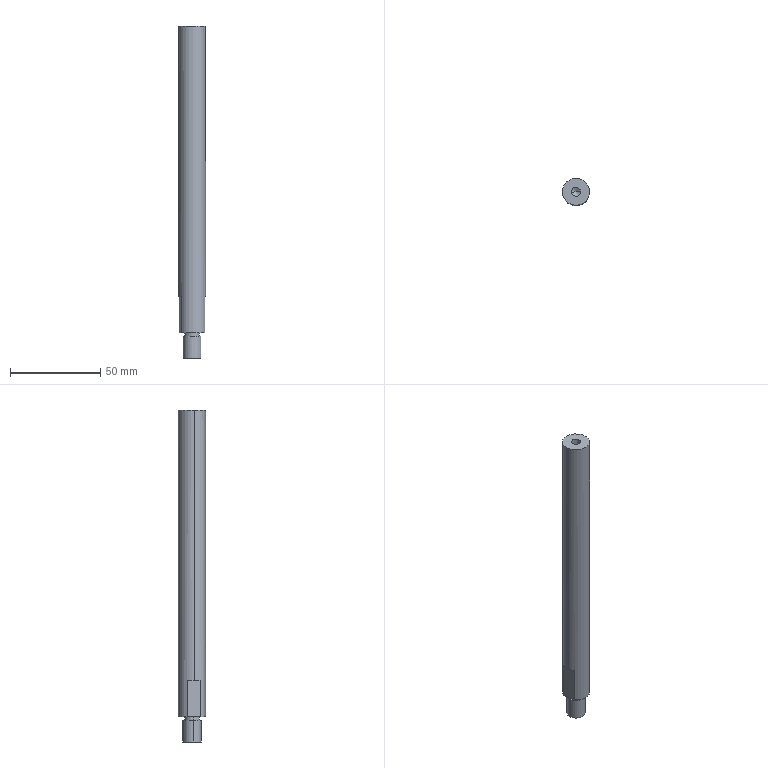Component | SolidWorks | -CoverTopPost-1 | 1 solid | 18 faces | box 15 x 15 x 184 mm | volume 30538 mm3 | cylinder 8 | plane 8 | cone 2 | commonest cylinder face diameters 10 x2 8 x2 5 x2 15 x2
build123d program:
from build123d import *

# Parameters (mm, degrees)
SKETCH1_R             = 7.5
BOSS_EXTRUDE1_DEPTH   = 85
M6_TAPPED_HOLE1_D     = 5
M6_TAPPED_HOLE1_DEPTH = 17
M6_TAPPED_HOLE1_TIP   = 1.502
SKETCH4_R             = 4
BOSS_EXTRUDE2_DEPTH   = 2
SKETCH5_R             = 5
BOSS_EXTRUDE3_DEPTH   = 12
SKETCH6_W             = 19.221
SKETCH6_H             = 36.695
SKETCH6_W_2           = 15.818
SKETCH6_H_2           = 41.018
CUT_EXTRUDE1_DEPTH    = 20


with BuildPart() as part:
    # Sketch1 → Boss-Extrude1 (new, symmetric)
    with BuildSketch(Plane.XY):
        Circle(SKETCH1_R)
    extrude(amount=BOSS_EXTRUDE1_DEPTH, both=True)

    # M6 Tapped Hole1
    with Locations(Plane.XY.offset(85)):
        with Locations((0, 0)):
            Hole(M6_TAPPED_HOLE1_D / 2, depth=M6_TAPPED_HOLE1_DEPTH)
            with Locations((0, 0, -(M6_TAPPED_HOLE1_DEPTH + M6_TAPPED_HOLE1_TIP / 2))):  # 118° drill point
                Cone(0, M6_TAPPED_HOLE1_D / 2, M6_TAPPED_HOLE1_TIP, mode=Mode.SUBTRACT)

    # Sketch4 → Boss-Extrude2 (add)
    with BuildSketch(Plane(origin=(0, 0, -85), x_dir=(-1, 0, 0), z_dir=(0, 0, -1))):
        with Locations(Location((0, 0, 0), (0, 0, 180))):
            Circle(SKETCH4_R)
    extrude(amount=BOSS_EXTRUDE2_DEPTH)

    # Sketch5 → Boss-Extrude3 (add)
    with BuildSketch(Plane(origin=(0, 0, -87), x_dir=(-1, 0, 0), z_dir=(0, 0, -1))):
        Circle(SKETCH5_R)
    extrude(amount=BOSS_EXTRUDE3_DEPTH)

    # Sketch6 → Cut-Extrude1 (cut)
    with BuildSketch(Plane(origin=(0, 0, -85), x_dir=(-1, 0, 0), z_dir=(0, 0, -1))):
        with Locations((-16.111, -0.5037)):
            Rectangle(SKETCH6_W, SKETCH6_H)
        with Locations((14.409, -0.5497)):
            Rectangle(SKETCH6_W_2, SKETCH6_H_2)
    extrude(amount=-CUT_EXTRUDE1_DEPTH, mode=Mode.SUBTRACT)


solid = part.part

# Placed as in the assembly
solid = solid.moved(Location((-15, 1079.5, 90), (0, 0, 9.293)))
STEP:
#1=COLOUR_RGB('',0.7922,0.8196,0.9333);
#2=FILL_AREA_STYLE_COLOUR('',#1);
#3=FILL_AREA_STYLE('',(#2));
#4=SURFACE_STYLE_FILL_AREA(#3);
#5=SURFACE_SIDE_STYLE('',(#4));
#6=SURFACE_STYLE_USAGE(.BOTH.,#5);
#7=PRESENTATION_STYLE_ASSIGNMENT((#6));
#8=CARTESIAN_POINT('',(-0.7848,42.468,-0.3543));
#9=VERTEX_POINT('',#8);
#10=CARTESIAN_POINT('',(-0.3963,42.532,-0.3543));
#11=VERTEX_POINT('',#10);
#12=CARTESIAN_POINT('',(-0.5906,42.5,-0.3543));
#13=DIRECTION('',(0.,0.,-1.));
#14=DIRECTION('',(-0.9869,-0.1615,0.));
#15=AXIS2_PLACEMENT_3D('',#12,#13,#14);
#16=CIRCLE('',#15,0.1969);
#17=EDGE_CURVE('',#9,#11,#16,.T.);
#18=ORIENTED_EDGE('',*,*,#17,.F.);
#19=CARTESIAN_POINT('',(-0.7848,42.468,0.1181));
#20=VERTEX_POINT('',#19);
#21=CARTESIAN_POINT('',(-0.7848,42.468,-0.3543));
#22=DIRECTION('',(0.,0.,1.));
#23=VECTOR('',#22,39.37);
#24=LINE('',#21,#23);
#25=EDGE_CURVE('',#9,#20,#24,.T.);
#26=ORIENTED_EDGE('',*,*,#25,.T.);
#27=CARTESIAN_POINT('',(-0.3963,42.532,0.1181));
#28=VERTEX_POINT('',#27);
#29=CARTESIAN_POINT('',(-0.5906,42.5,0.1181));
#30=DIRECTION('',(0.,0.,-1.));
#31=DIRECTION('',(-0.9869,-0.1615,0.));
#32=AXIS2_PLACEMENT_3D('',#29,#30,#31);
#33=CIRCLE('',#32,0.1969);
#34=EDGE_CURVE('',#20,#28,#33,.T.);
#35=ORIENTED_EDGE('',*,*,#34,.T.);
#36=CARTESIAN_POINT('',(-0.3963,42.532,-0.3543));
#37=DIRECTION('',(0.,0.,1.));
#38=VECTOR('',#37,39.37);
#39=LINE('',#36,#38);
#40=EDGE_CURVE('',#11,#28,#39,.T.);
#41=ORIENTED_EDGE('',*,*,#40,.F.);
#42=EDGE_LOOP('',(#18,#26,#35,#41));
#43=FACE_OUTER_BOUND('',#42,.T.);
#44=CARTESIAN_POINT('',(-0.5906,42.5,-0.3543));
#45=DIRECTION('',(0.,0.,1.));
#46=DIRECTION('',(0.9869,0.1615,0.));
#47=AXIS2_PLACEMENT_3D('',#44,#45,#46);
#48=CYLINDRICAL_SURFACE('',#47,0.1969);
#49=ADVANCED_FACE('',(#43),#48,.T.);
#50=CARTESIAN_POINT('',(-0.746,42.475,0.1181));
#51=VERTEX_POINT('',#50);
#52=CARTESIAN_POINT('',(-0.4351,42.525,0.1181));
#53=VERTEX_POINT('',#52);
#54=CARTESIAN_POINT('',(-0.5906,42.5,0.1181));
#55=DIRECTION('',(0.,0.,-1.));
#56=DIRECTION('',(-0.9869,-0.1615,0.));
#57=AXIS2_PLACEMENT_3D('',#54,#55,#56);
#58=CIRCLE('',#57,0.1575);
#59=EDGE_CURVE('',#51,#53,#58,.T.);
#60=ORIENTED_EDGE('',*,*,#59,.F.);
#61=CARTESIAN_POINT('',(-0.746,42.475,0.1969));
#62=VERTEX_POINT('',#61);
#63=CARTESIAN_POINT('',(-0.746,42.475,0.1181));
#64=DIRECTION('',(0.,0.,1.));
#65=VECTOR('',#64,39.37);
#66=LINE('',#63,#65);
#67=EDGE_CURVE('',#51,#62,#66,.T.);
#68=ORIENTED_EDGE('',*,*,#67,.T.);
#69=CARTESIAN_POINT('',(-0.4351,42.525,0.1969));
#70=VERTEX_POINT('',#69);
#71=CARTESIAN_POINT('',(-0.5906,42.5,0.1969));
#72=DIRECTION('',(0.,0.,-1.));
#73=DIRECTION('',(0.9869,0.1615,0.));
#74=AXIS2_PLACEMENT_3D('',#71,#72,#73);
#75=CIRCLE('',#74,0.1575);
#76=EDGE_CURVE('',#62,#70,#75,.T.);
#77=ORIENTED_EDGE('',*,*,#76,.T.);
#78=CARTESIAN_POINT('',(-0.4351,42.525,0.1181));
#79=DIRECTION('',(0.,0.,1.));
#80=VECTOR('',#79,39.37);
#81=LINE('',#78,#80);
#82=EDGE_CURVE('',#53,#70,#81,.T.);
#83=ORIENTED_EDGE('',*,*,#82,.F.);
#84=EDGE_LOOP('',(#60,#68,#77,#83));
#85=FACE_OUTER_BOUND('',#84,.T.);
#86=CARTESIAN_POINT('',(-0.5906,42.5,0.1181));
#87=DIRECTION('',(0.,0.,1.));
#88=DIRECTION('',(0.9869,0.1615,0.));
#89=AXIS2_PLACEMENT_3D('',#86,#87,#88);
#90=CYLINDRICAL_SURFACE('',#89,0.1575);
#91=ADVANCED_FACE('',(#85),#90,.T.);
#92=CARTESIAN_POINT('',(-0.6877,42.484,6.22));
#93=VERTEX_POINT('',#92);
#94=CARTESIAN_POINT('',(-0.4934,42.516,6.22));
#95=VERTEX_POINT('',#94);
#96=CARTESIAN_POINT('',(-0.5906,42.5,6.22));
#97=DIRECTION('',(0.,0.,1.));
#98=DIRECTION('',(0.9869,0.1615,0.));
#99=AXIS2_PLACEMENT_3D('',#96,#97,#98);
#100=CIRCLE('',#99,0.09843);
#101=EDGE_CURVE('',#93,#95,#100,.T.);
#102=ORIENTED_EDGE('',*,*,#101,.F.);
#103=CARTESIAN_POINT('',(-0.6877,42.484,6.89));
#104=VERTEX_POINT('',#103);
#105=CARTESIAN_POINT('',(-0.6877,42.484,6.89));
#106=DIRECTION('',(0.,0.,1.));
#107=VECTOR('',#106,39.37);
#108=LINE('',#105,#107);
#109=EDGE_CURVE('',#93,#104,#108,.T.);
#110=ORIENTED_EDGE('',*,*,#109,.T.);
#111=CARTESIAN_POINT('',(-0.4934,42.516,6.89));
#112=VERTEX_POINT('',#111);
#113=CARTESIAN_POINT('',(-0.5906,42.5,6.89));
#114=DIRECTION('',(0.,0.,1.));
#115=DIRECTION('',(0.9869,0.1615,0.));
#116=AXIS2_PLACEMENT_3D('',#113,#114,#115);
#117=CIRCLE('',#116,0.09843);
#118=EDGE_CURVE('',#104,#112,#117,.T.);
#119=ORIENTED_EDGE('',*,*,#118,.T.);
#120=CARTESIAN_POINT('',(-0.4934,42.516,6.89));
#121=DIRECTION('',(0.,0.,1.));
#122=VECTOR('',#121,39.37);
#123=LINE('',#120,#122);
#124=EDGE_CURVE('',#95,#112,#123,.T.);
#125=ORIENTED_EDGE('',*,*,#124,.F.);
#126=EDGE_LOOP('',(#102,#110,#119,#125));
#127=FACE_OUTER_BOUND('',#126,.T.);
#128=CARTESIAN_POINT('',(-0.5906,42.5,6.89));
#129=DIRECTION('',(0.,0.,1.));
#130=DIRECTION('',(0.9869,0.1615,0.));
#131=AXIS2_PLACEMENT_3D('',#128,#129,#130);
#132=CYLINDRICAL_SURFACE('',#131,0.09843);
#133=ADVANCED_FACE('',(#127),#132,.F.);
#134=CARTESIAN_POINT('',(-0.5906,42.5,6.161));
#135=VERTEX_POINT('',#134);
#136=CARTESIAN_POINT('',(-0.4934,42.516,6.22));
#137=DIRECTION('',(0.8459,0.1384,0.515));
#138=VECTOR('',#137,39.37);
#139=LINE('',#136,#138);
#140=EDGE_CURVE('',#135,#95,#139,.T.);
#141=ORIENTED_EDGE('',*,*,#140,.F.);
#142=CARTESIAN_POINT('',(-0.6877,42.484,6.22));
#143=DIRECTION('',(-0.8459,-0.1384,0.515));
#144=VECTOR('',#143,39.37);
#145=LINE('',#142,#144);
#146=EDGE_CURVE('',#135,#93,#145,.T.);
#147=ORIENTED_EDGE('',*,*,#146,.T.);
#148=ORIENTED_EDGE('',*,*,#101,.T.);
#149=EDGE_LOOP('',(#141,#147,#148));
#150=FACE_OUTER_BOUND('',#149,.T.);
#151=CARTESIAN_POINT('',(-0.5906,42.5,6.22));
#152=DIRECTION('',(0.,0.,1.));
#153=DIRECTION('',(0.9869,0.1615,0.));
#154=AXIS2_PLACEMENT_3D('',#151,#152,#153);
#155=CONICAL_SURFACE('',#154,0.09843,1.03);
#156=ADVANCED_FACE('',(#150),#155,.F.);
#157=CARTESIAN_POINT('',(-0.2992,42.548,6.89));
#158=VERTEX_POINT('',#157);
#159=CARTESIAN_POINT('',(-0.882,42.452,6.89));
#160=VERTEX_POINT('',#159);
#161=CARTESIAN_POINT('',(-0.5906,42.5,6.89));
#162=DIRECTION('',(0.,0.,1.));
#163=DIRECTION('',(0.9869,0.1615,0.));
#164=AXIS2_PLACEMENT_3D('',#161,#162,#163);
#165=CIRCLE('',#164,0.2953);
#166=EDGE_CURVE('',#158,#160,#165,.T.);
#167=ORIENTED_EDGE('',*,*,#166,.F.);
#168=CARTESIAN_POINT('',(-0.2992,42.548,0.9843));
#169=VERTEX_POINT('',#168);
#170=CARTESIAN_POINT('',(-0.2992,42.548,6.89));
#171=DIRECTION('',(0.,0.,-1.));
#172=VECTOR('',#171,39.37);
#173=LINE('',#170,#172);
#174=EDGE_CURVE('',#158,#169,#173,.T.);
#175=ORIENTED_EDGE('',*,*,#174,.T.);
#176=CARTESIAN_POINT('',(-0.3618,42.687,0.9843));
#177=VERTEX_POINT('',#176);
#178=CARTESIAN_POINT('',(-0.5906,42.5,0.9843));
#179=DIRECTION('',(0.,0.,-1.));
#180=DIRECTION('',(-0.9869,-0.1615,0.));
#181=AXIS2_PLACEMENT_3D('',#178,#179,#180);
#182=CIRCLE('',#181,0.2953);
#183=EDGE_CURVE('',#177,#169,#182,.T.);
#184=ORIENTED_EDGE('',*,*,#183,.F.);
#185=CARTESIAN_POINT('',(-0.3618,42.687,0.1969));
#186=VERTEX_POINT('',#185);
#187=CARTESIAN_POINT('',(-0.3618,42.687,6.89));
#188=DIRECTION('',(0.,0.,-1.));
#189=VECTOR('',#188,39.37);
#190=LINE('',#187,#189);
#191=EDGE_CURVE('',#177,#186,#190,.T.);
#192=ORIENTED_EDGE('',*,*,#191,.T.);
#193=CARTESIAN_POINT('',(-0.8669,42.604,0.1969));
#194=VERTEX_POINT('',#193);
#195=CARTESIAN_POINT('',(-0.5906,42.5,0.1969));
#196=DIRECTION('',(0.,0.,1.));
#197=DIRECTION('',(0.9869,0.1615,0.));
#198=AXIS2_PLACEMENT_3D('',#195,#196,#197);
#199=CIRCLE('',#198,0.2953);
#200=EDGE_CURVE('',#186,#194,#199,.T.);
#201=ORIENTED_EDGE('',*,*,#200,.T.);
#202=CARTESIAN_POINT('',(-0.8669,42.604,0.9843));
#203=VERTEX_POINT('',#202);
#204=CARTESIAN_POINT('',(-0.8669,42.604,6.89));
#205=DIRECTION('',(0.,0.,1.));
#206=VECTOR('',#205,39.37);
#207=LINE('',#204,#206);
#208=EDGE_CURVE('',#194,#203,#207,.T.);
#209=ORIENTED_EDGE('',*,*,#208,.T.);
#210=CARTESIAN_POINT('',(-0.882,42.452,0.9843));
#211=VERTEX_POINT('',#210);
#212=CARTESIAN_POINT('',(-0.5906,42.5,0.9843));
#213=DIRECTION('',(0.,0.,1.));
#214=DIRECTION('',(0.9869,0.1615,0.));
#215=AXIS2_PLACEMENT_3D('',#212,#213,#214);
#216=CIRCLE('',#215,0.2953);
#217=EDGE_CURVE('',#203,#211,#216,.T.);
#218=ORIENTED_EDGE('',*,*,#217,.T.);
#219=CARTESIAN_POINT('',(-0.882,42.452,6.89));
#220=DIRECTION('',(0.,0.,-1.));
#221=VECTOR('',#220,39.37);
#222=LINE('',#219,#221);
#223=EDGE_CURVE('',#160,#211,#222,.T.);
#224=ORIENTED_EDGE('',*,*,#223,.F.);
#225=EDGE_LOOP('',(#167,#175,#184,#192,#201,#209,#218,#224));
#226=FACE_OUTER_BOUND('',#225,.T.);
#227=CARTESIAN_POINT('',(-0.5906,42.5,6.89));
#228=DIRECTION('',(0.,0.,-1.));
#229=DIRECTION('',(-0.9869,-0.1615,0.));
#230=AXIS2_PLACEMENT_3D('',#227,#228,#229);
#231=CYLINDRICAL_SURFACE('',#230,0.2953);
#232=ADVANCED_FACE('',(#226),#231,.T.);
#233=CARTESIAN_POINT('',(-0.8193,42.313,0.1969));
#234=VERTEX_POINT('',#233);
#235=CARTESIAN_POINT('',(-0.3142,42.396,0.1969));
#236=VERTEX_POINT('',#235);
#237=CARTESIAN_POINT('',(-0.5906,42.5,0.1969));
#238=DIRECTION('',(0.,0.,1.));
#239=DIRECTION('',(0.9869,0.1615,0.));
#240=AXIS2_PLACEMENT_3D('',#237,#238,#239);
#241=CIRCLE('',#240,0.2953);
#242=EDGE_CURVE('',#234,#236,#241,.T.);
#243=ORIENTED_EDGE('',*,*,#242,.F.);
#244=CARTESIAN_POINT('',(-0.97,43.234,0.1969));
#245=DIRECTION('',(0.1615,-0.9869,0.));
#246=VECTOR('',#245,39.37);
#247=LINE('',#244,#246);
#248=EDGE_CURVE('',#194,#234,#247,.T.);
#249=ORIENTED_EDGE('',*,*,#248,.F.);
#250=ORIENTED_EDGE('',*,*,#200,.F.);
#251=CARTESIAN_POINT('',(-0.4514,43.235,0.1969));
#252=DIRECTION('',(-0.1615,0.9869,0.));
#253=VECTOR('',#252,39.37);
#254=LINE('',#251,#253);
#255=EDGE_CURVE('',#236,#186,#254,.T.);
#256=ORIENTED_EDGE('',*,*,#255,.F.);
#257=EDGE_LOOP('',(#243,#249,#250,#256));
#258=FACE_OUTER_BOUND('',#257,.T.);
#259=CARTESIAN_POINT('',(-0.5906,42.5,0.1969));
#260=DIRECTION('',(0.,0.,-1.));
#261=DIRECTION('',(0.9869,0.1615,0.));
#262=AXIS2_PLACEMENT_3D('',#259,#260,#261);
#263=CIRCLE('',#262,0.1575);
#264=EDGE_CURVE('',#70,#62,#263,.T.);
#265=ORIENTED_EDGE('',*,*,#264,.F.);
#266=ORIENTED_EDGE('',*,*,#76,.F.);
#267=EDGE_LOOP('',(#265,#266));
#268=FACE_BOUND('',#267,.T.);
#269=CARTESIAN_POINT('',(-0.5906,42.5,0.1969));
#270=DIRECTION('',(0.,0.,1.));
#271=DIRECTION('',(0.9869,0.1615,0.));
#272=AXIS2_PLACEMENT_3D('',#269,#270,#271);
#273=PLANE('',#272);
#274=ADVANCED_FACE('',(#258,#268),#273,.F.);
#275=ORIENTED_EDGE('',*,*,#174,.F.);
#276=CARTESIAN_POINT('',(-0.5906,42.5,6.89));
#277=DIRECTION('',(0.,0.,1.));
#278=DIRECTION('',(0.9869,0.1615,0.));
#279=AXIS2_PLACEMENT_3D('',#276,#277,#278);
#280=CIRCLE('',#279,0.2953);
#281=EDGE_CURVE('',#160,#158,#280,.T.);
#282=ORIENTED_EDGE('',*,*,#281,.F.);
#283=ORIENTED_EDGE('',*,*,#223,.T.);
#284=CARTESIAN_POINT('',(-0.8193,42.313,0.9843));
#285=VERTEX_POINT('',#284);
#286=CARTESIAN_POINT('',(-0.5906,42.5,0.9843));
#287=DIRECTION('',(0.,0.,1.));
#288=DIRECTION('',(0.9869,0.1615,0.));
#289=AXIS2_PLACEMENT_3D('',#286,#287,#288);
#290=CIRCLE('',#289,0.2953);
#291=EDGE_CURVE('',#211,#285,#290,.T.);
#292=ORIENTED_EDGE('',*,*,#291,.T.);
#293=CARTESIAN_POINT('',(-0.8193,42.313,6.89));
#294=DIRECTION('',(0.,0.,-1.));
#295=VECTOR('',#294,39.37);
#296=LINE('',#293,#295);
#297=EDGE_CURVE('',#285,#234,#296,.T.);
#298=ORIENTED_EDGE('',*,*,#297,.T.);
#299=ORIENTED_EDGE('',*,*,#242,.T.);
#300=CARTESIAN_POINT('',(-0.3142,42.396,0.9843));
#301=VERTEX_POINT('',#300);
#302=CARTESIAN_POINT('',(-0.3142,42.396,6.89));
#303=DIRECTION('',(0.,0.,1.));
#304=VECTOR('',#303,39.37);
#305=LINE('',#302,#304);
#306=EDGE_CURVE('',#236,#301,#305,.T.);
#307=ORIENTED_EDGE('',*,*,#306,.T.);
#308=CARTESIAN_POINT('',(-0.5906,42.5,0.9843));
#309=DIRECTION('',(0.,0.,-1.));
#310=DIRECTION('',(-0.9869,-0.1615,0.));
#311=AXIS2_PLACEMENT_3D('',#308,#309,#310);
#312=CIRCLE('',#311,0.2953);
#313=EDGE_CURVE('',#169,#301,#312,.T.);
#314=ORIENTED_EDGE('',*,*,#313,.F.);
#315=EDGE_LOOP('',(#275,#282,#283,#292,#298,#299,#307,#314));
#316=FACE_OUTER_BOUND('',#315,.T.);
#317=CARTESIAN_POINT('',(-0.5906,42.5,6.89));
#318=DIRECTION('',(0.,0.,-1.));
#319=DIRECTION('',(-0.9869,-0.1615,0.));
#320=AXIS2_PLACEMENT_3D('',#317,#318,#319);
#321=CYLINDRICAL_SURFACE('',#320,0.2953);
#322=ADVANCED_FACE('',(#316),#321,.T.);
#323=CARTESIAN_POINT('',(-0.5906,42.5,6.89));
#324=DIRECTION('',(0.,0.,1.));
#325=DIRECTION('',(0.9869,0.1615,0.));
#326=AXIS2_PLACEMENT_3D('',#323,#324,#325);
#327=CIRCLE('',#326,0.09843);
#328=EDGE_CURVE('',#112,#104,#327,.T.);
#329=ORIENTED_EDGE('',*,*,#328,.F.);
#330=ORIENTED_EDGE('',*,*,#118,.F.);
#331=EDGE_LOOP('',(#329,#330));
#332=FACE_BOUND('',#331,.T.);
#333=ORIENTED_EDGE('',*,*,#281,.T.);
#334=ORIENTED_EDGE('',*,*,#166,.T.);
#335=EDGE_LOOP('',(#333,#334));
#336=FACE_OUTER_BOUND('',#335,.T.);
#337=CARTESIAN_POINT('',(-0.5906,42.5,6.89));
#338=DIRECTION('',(0.,0.,1.));
#339=DIRECTION('',(0.9869,0.1615,0.));
#340=AXIS2_PLACEMENT_3D('',#337,#338,#339);
#341=PLANE('',#340);
#342=ADVANCED_FACE('',(#332,#336),#341,.T.);
#343=ORIENTED_EDGE('',*,*,#146,.F.);
#344=ORIENTED_EDGE('',*,*,#140,.T.);
#345=CARTESIAN_POINT('',(-0.5906,42.5,6.22));
#346=DIRECTION('',(0.,0.,1.));
#347=DIRECTION('',(0.9869,0.1615,0.));
#348=AXIS2_PLACEMENT_3D('',#345,#346,#347);
#349=CIRCLE('',#348,0.09843);
#350=EDGE_CURVE('',#95,#93,#349,.T.);
#351=ORIENTED_EDGE('',*,*,#350,.T.);
#352=EDGE_LOOP('',(#343,#344,#351));
#353=FACE_OUTER_BOUND('',#352,.T.);
#354=CARTESIAN_POINT('',(-0.5906,42.5,6.22));
#355=DIRECTION('',(0.,0.,1.));
#356=DIRECTION('',(0.9869,0.1615,0.));
#357=AXIS2_PLACEMENT_3D('',#354,#355,#356);
#358=CONICAL_SURFACE('',#357,0.09843,1.03);
#359=ADVANCED_FACE('',(#353),#358,.F.);
#360=ORIENTED_EDGE('',*,*,#109,.F.);
#361=ORIENTED_EDGE('',*,*,#350,.F.);
#362=ORIENTED_EDGE('',*,*,#124,.T.);
#363=ORIENTED_EDGE('',*,*,#328,.T.);
#364=EDGE_LOOP('',(#360,#361,#362,#363));
#365=FACE_OUTER_BOUND('',#364,.T.);
#366=CARTESIAN_POINT('',(-0.5906,42.5,6.89));
#367=DIRECTION('',(0.,0.,1.));
#368=DIRECTION('',(0.9869,0.1615,0.));
#369=AXIS2_PLACEMENT_3D('',#366,#367,#368);
#370=CYLINDRICAL_SURFACE('',#369,0.09843);
#371=ADVANCED_FACE('',(#365),#370,.F.);
#372=ORIENTED_EDGE('',*,*,#67,.F.);
#373=CARTESIAN_POINT('',(-0.5906,42.5,0.1181));
#374=DIRECTION('',(0.,0.,-1.));
#375=DIRECTION('',(-0.9869,-0.1615,0.));
#376=AXIS2_PLACEMENT_3D('',#373,#374,#375);
#377=CIRCLE('',#376,0.1575);
#378=EDGE_CURVE('',#53,#51,#377,.T.);
#379=ORIENTED_EDGE('',*,*,#378,.F.);
#380=ORIENTED_EDGE('',*,*,#82,.T.);
#381=ORIENTED_EDGE('',*,*,#264,.T.);
#382=EDGE_LOOP('',(#372,#379,#380,#381));
#383=FACE_OUTER_BOUND('',#382,.T.);
#384=CARTESIAN_POINT('',(-0.5906,42.5,0.1181));
#385=DIRECTION('',(0.,0.,1.));
#386=DIRECTION('',(0.9869,0.1615,0.));
#387=AXIS2_PLACEMENT_3D('',#384,#385,#386);
#388=CYLINDRICAL_SURFACE('',#387,0.1575);
#389=ADVANCED_FACE('',(#383),#388,.T.);
#390=CARTESIAN_POINT('',(-0.5906,42.5,0.1181));
#391=DIRECTION('',(0.,0.,-1.));
#392=DIRECTION('',(-0.9869,-0.1615,0.));
#393=AXIS2_PLACEMENT_3D('',#390,#391,#392);
#394=CIRCLE('',#393,0.1969);
#395=EDGE_CURVE('',#28,#20,#394,.T.);
#396=ORIENTED_EDGE('',*,*,#395,.F.);
#397=ORIENTED_EDGE('',*,*,#34,.F.);
#398=EDGE_LOOP('',(#396,#397));
#399=FACE_OUTER_BOUND('',#398,.T.);
#400=ORIENTED_EDGE('',*,*,#378,.T.);
#401=ORIENTED_EDGE('',*,*,#59,.T.);
#402=EDGE_LOOP('',(#400,#401));
#403=FACE_BOUND('',#402,.T.);
#404=CARTESIAN_POINT('',(-0.5906,42.5,0.1181));
#405=DIRECTION('',(0.,0.,-1.));
#406=DIRECTION('',(-0.9869,-0.1615,0.));
#407=AXIS2_PLACEMENT_3D('',#404,#405,#406);
#408=PLANE('',#407);
#409=ADVANCED_FACE('',(#399,#403),#408,.F.);
#410=ORIENTED_EDGE('',*,*,#25,.F.);
#411=CARTESIAN_POINT('',(-0.5906,42.5,-0.3543));
#412=DIRECTION('',(0.,0.,-1.));
#413=DIRECTION('',(-0.9869,-0.1615,0.));
#414=AXIS2_PLACEMENT_3D('',#411,#412,#413);
#415=CIRCLE('',#414,0.1969);
#416=EDGE_CURVE('',#11,#9,#415,.T.);
#417=ORIENTED_EDGE('',*,*,#416,.F.);
#418=ORIENTED_EDGE('',*,*,#40,.T.);
#419=ORIENTED_EDGE('',*,*,#395,.T.);
#420=EDGE_LOOP('',(#410,#417,#418,#419));
#421=FACE_OUTER_BOUND('',#420,.T.);
#422=CARTESIAN_POINT('',(-0.5906,42.5,-0.3543));
#423=DIRECTION('',(0.,0.,1.));
#424=DIRECTION('',(0.9869,0.1615,0.));
#425=AXIS2_PLACEMENT_3D('',#422,#423,#424);
#426=CYLINDRICAL_SURFACE('',#425,0.1969);
#427=ADVANCED_FACE('',(#421),#426,.T.);
#428=ORIENTED_EDGE('',*,*,#416,.T.);
#429=ORIENTED_EDGE('',*,*,#17,.T.);
#430=EDGE_LOOP('',(#428,#429));
#431=FACE_OUTER_BOUND('',#430,.T.);
#432=CARTESIAN_POINT('',(-0.5906,42.5,-0.3543));
#433=DIRECTION('',(0.,0.,-1.));
#434=DIRECTION('',(-0.9869,-0.1615,0.));
#435=AXIS2_PLACEMENT_3D('',#432,#433,#434);
#436=PLANE('',#435);
#437=ADVANCED_FACE('',(#431),#436,.T.);
#438=CARTESIAN_POINT('',(-0.4514,43.235,0.9843));
#439=DIRECTION('',(-0.1615,0.9869,0.));
#440=VECTOR('',#439,39.37);
#441=LINE('',#438,#440);
#442=EDGE_CURVE('',#301,#177,#441,.T.);
#443=ORIENTED_EDGE('',*,*,#442,.F.);
#444=ORIENTED_EDGE('',*,*,#306,.F.);
#445=ORIENTED_EDGE('',*,*,#255,.T.);
#446=ORIENTED_EDGE('',*,*,#191,.F.);
#447=EDGE_LOOP('',(#443,#444,#445,#446));
#448=FACE_OUTER_BOUND('',#447,.T.);
#449=CARTESIAN_POINT('',(-0.4514,43.235,0.9843));
#450=DIRECTION('',(-0.9869,-0.1615,0.));
#451=DIRECTION('',(0.1615,-0.9869,0.));
#452=AXIS2_PLACEMENT_3D('',#449,#450,#451);
#453=PLANE('',#452);
#454=ADVANCED_FACE('',(#448),#453,.F.);
#455=ORIENTED_EDGE('',*,*,#183,.T.);
#456=ORIENTED_EDGE('',*,*,#313,.T.);
#457=ORIENTED_EDGE('',*,*,#442,.T.);
#458=EDGE_LOOP('',(#455,#456,#457));
#459=FACE_OUTER_BOUND('',#458,.T.);
#460=CARTESIAN_POINT('',(-0.5906,42.5,0.9843));
#461=DIRECTION('',(0.,0.,-1.));
#462=DIRECTION('',(-0.9869,-0.1615,0.));
#463=AXIS2_PLACEMENT_3D('',#460,#461,#462);
#464=PLANE('',#463);
#465=ADVANCED_FACE('',(#459),#464,.T.);
#466=CARTESIAN_POINT('',(-0.97,43.234,0.9843));
#467=DIRECTION('',(0.1615,-0.9869,0.));
#468=VECTOR('',#467,39.37);
#469=LINE('',#466,#468);
#470=EDGE_CURVE('',#203,#285,#469,.T.);
#471=ORIENTED_EDGE('',*,*,#470,.F.);
#472=ORIENTED_EDGE('',*,*,#208,.F.);
#473=ORIENTED_EDGE('',*,*,#248,.T.);
#474=ORIENTED_EDGE('',*,*,#297,.F.);
#475=EDGE_LOOP('',(#471,#472,#473,#474));
#476=FACE_OUTER_BOUND('',#475,.T.);
#477=CARTESIAN_POINT('',(-0.97,43.234,0.9843));
#478=DIRECTION('',(0.9869,0.1615,0.));
#479=DIRECTION('',(-0.1615,0.9869,0.));
#480=AXIS2_PLACEMENT_3D('',#477,#478,#479);
#481=PLANE('',#480);
#482=ADVANCED_FACE('',(#476),#481,.F.);
#483=ORIENTED_EDGE('',*,*,#470,.T.);
#484=ORIENTED_EDGE('',*,*,#291,.F.);
#485=ORIENTED_EDGE('',*,*,#217,.F.);
#486=EDGE_LOOP('',(#483,#484,#485));
#487=FACE_OUTER_BOUND('',#486,.T.);
#488=CARTESIAN_POINT('',(-0.5906,42.5,0.9843));
#489=DIRECTION('',(0.,0.,1.));
#490=DIRECTION('',(0.9869,0.1615,0.));
#491=AXIS2_PLACEMENT_3D('',#488,#489,#490);
#492=PLANE('',#491);
#493=ADVANCED_FACE('',(#487),#492,.F.);
#494=CLOSED_SHELL('',(#49,#91,#133,#156,#232,#274,#322,#342,#359,#371,#389,#409,#427,#437,#454,#465,#482,#493));
#495=MANIFOLD_SOLID_BREP('',#494);
#496=STYLED_ITEM('',(#7),#495);
#497=PRESENTATION_LAYER_ASSIGNMENT('','',(#496));
#498=(LENGTH_UNIT()NAMED_UNIT(*)SI_UNIT($,.METRE.));
#499=LENGTH_MEASURE_WITH_UNIT(LENGTH_MEASURE(0.0254),#498);
#500=DIMENSIONAL_EXPONENTS(1.,0.,0.,0.,0.,0.,0.);
#501=(CONVERSION_BASED_UNIT('',#499)LENGTH_UNIT()NAMED_UNIT(#500));
#502=UNCERTAINTY_MEASURE_WITH_UNIT(LENGTH_MEASURE(0.00001),#501,'','');
#503=(NAMED_UNIT(*)PLANE_ANGLE_UNIT()SI_UNIT($,.RADIAN.));
#504=(NAMED_UNIT(*)SI_UNIT($,.STERADIAN.)SOLID_ANGLE_UNIT());
#505=(GEOMETRIC_REPRESENTATION_CONTEXT(3)GLOBAL_UNCERTAINTY_ASSIGNED_CONTEXT((#502))GLOBAL_UNIT_ASSIGNED_CONTEXT((#501,#503,#504))REPRESENTATION_CONTEXT('',''));
#506=MECHANICAL_DESIGN_GEOMETRIC_PRESENTATION_REPRESENTATION('',(#496),#505);
#507=CARTESIAN_POINT('',(0.,0.,0.));
#508=DIRECTION('',(0.,0.,1.));
#509=DIRECTION('',(1.,0.,0.));
#510=AXIS2_PLACEMENT_3D('',#507,#508,#509);
#511=(LENGTH_UNIT()NAMED_UNIT(*)SI_UNIT($,.METRE.));
#512=LENGTH_MEASURE_WITH_UNIT(LENGTH_MEASURE(0.0254),#511);
#513=DIMENSIONAL_EXPONENTS(1.,0.,0.,0.,0.,0.,0.);
#514=(CONVERSION_BASED_UNIT('',#512)LENGTH_UNIT()NAMED_UNIT(#513));
#515=UNCERTAINTY_MEASURE_WITH_UNIT(LENGTH_MEASURE(0.00001),#514,'','');
#516=(NAMED_UNIT(*)PLANE_ANGLE_UNIT()SI_UNIT($,.RADIAN.));
#517=(NAMED_UNIT(*)SI_UNIT($,.STERADIAN.)SOLID_ANGLE_UNIT());
#518=(GEOMETRIC_REPRESENTATION_CONTEXT(3)GLOBAL_UNCERTAINTY_ASSIGNED_CONTEXT((#515))GLOBAL_UNIT_ASSIGNED_CONTEXT((#514,#516,#517))REPRESENTATION_CONTEXT('',''));
#519=ADVANCED_BREP_SHAPE_REPRESENTATION('',(#495,#510),#518);